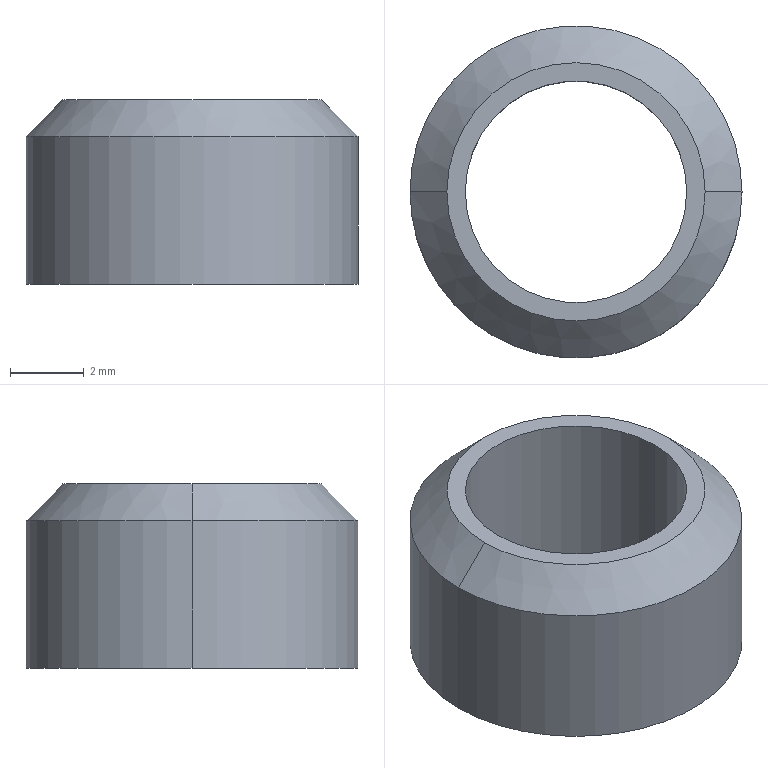Component | SolidWorks | Adjuster-1 | 1 solid | 8 faces | box 9 x 9 x 5 mm | volume 164 mm3 | cylinder 4 | cone 2 | plane 2 | commonest cylinder face diameters 6 x2 9 x2
build123d program:
from build123d import *

# Parameters (mm, degrees)
SKETCH1_R           = 4.5
SKETCH1_R_2         = 3
BOSS_EXTRUDE1_DEPTH = 5
CHAMFER1_SIZE       = 1


with BuildPart() as part:
    # Sketch1 → Boss-Extrude1 (new body)
    with BuildSketch(Plane.XY):
        Circle(SKETCH1_R)
        Circle(SKETCH1_R_2, mode=Mode.SUBTRACT)
    extrude(amount=BOSS_EXTRUDE1_DEPTH)

    # Chamfer1
    chamfer1_edges = [part.edges().sort_by_distance(p)[0] for p in [
        (-4.5, 0, 5),
    ]]
    chamfer(chamfer1_edges, length=CHAMFER1_SIZE)


solid = part.part

# Placed as in the assembly
solid = solid.moved(Location((-218.606, 95.367, 1090.85), (0, 0, 0)))
STEP:
#1=COLOUR_RGB('',0.7922,0.8196,0.9333);
#2=FILL_AREA_STYLE_COLOUR('',#1);
#3=FILL_AREA_STYLE('',(#2));
#4=SURFACE_STYLE_FILL_AREA(#3);
#5=SURFACE_SIDE_STYLE('',(#4));
#6=SURFACE_STYLE_USAGE(.BOTH.,#5);
#7=PRESENTATION_STYLE_ASSIGNMENT((#6));
#8=CARTESIAN_POINT('',(-8.469,3.755,43.144));
#9=VERTEX_POINT('',#8);
#10=CARTESIAN_POINT('',(-8.744,3.755,43.144));
#11=VERTEX_POINT('',#10);
#12=CARTESIAN_POINT('',(-8.607,3.755,43.144));
#13=DIRECTION('',(0.,0.,1.));
#14=DIRECTION('',(1.,0.,0.));
#15=AXIS2_PLACEMENT_3D('',#12,#13,#14);
#16=CIRCLE('',#15,0.1378);
#17=EDGE_CURVE('',#9,#11,#16,.T.);
#18=ORIENTED_EDGE('',*,*,#17,.F.);
#19=CARTESIAN_POINT('',(-8.429,3.755,43.104));
#20=VERTEX_POINT('',#19);
#21=CARTESIAN_POINT('',(-8.469,3.755,43.144));
#22=DIRECTION('',(0.7071,0.,-0.7071));
#23=VECTOR('',#22,39.37);
#24=LINE('',#21,#23);
#25=EDGE_CURVE('',#9,#20,#24,.T.);
#26=ORIENTED_EDGE('',*,*,#25,.T.);
#27=CARTESIAN_POINT('',(-8.784,3.755,43.104));
#28=VERTEX_POINT('',#27);
#29=CARTESIAN_POINT('',(-8.607,3.755,43.104));
#30=DIRECTION('',(0.,0.,-1.));
#31=DIRECTION('',(1.,0.,0.));
#32=AXIS2_PLACEMENT_3D('',#29,#30,#31);
#33=CIRCLE('',#32,0.1772);
#34=EDGE_CURVE('',#28,#20,#33,.T.);
#35=ORIENTED_EDGE('',*,*,#34,.F.);
#36=CARTESIAN_POINT('',(-8.744,3.755,43.144));
#37=DIRECTION('',(-0.7071,0.,-0.7071));
#38=VECTOR('',#37,39.37);
#39=LINE('',#36,#38);
#40=EDGE_CURVE('',#11,#28,#39,.T.);
#41=ORIENTED_EDGE('',*,*,#40,.F.);
#42=EDGE_LOOP('',(#18,#26,#35,#41));
#43=FACE_OUTER_BOUND('',#42,.T.);
#44=CARTESIAN_POINT('',(-8.607,3.755,43.144));
#45=DIRECTION('',(0.,0.,-1.));
#46=DIRECTION('',(-1.,0.,0.));
#47=AXIS2_PLACEMENT_3D('',#44,#45,#46);
#48=CONICAL_SURFACE('',#47,0.1378,0.7854);
#49=ADVANCED_FACE('',(#43),#48,.T.);
#50=CARTESIAN_POINT('',(-8.725,3.755,43.144));
#51=VERTEX_POINT('',#50);
#52=CARTESIAN_POINT('',(-8.488,3.755,43.144));
#53=VERTEX_POINT('',#52);
#54=CARTESIAN_POINT('',(-8.607,3.755,43.144));
#55=DIRECTION('',(0.,0.,1.));
#56=DIRECTION('',(1.,0.,0.));
#57=AXIS2_PLACEMENT_3D('',#54,#55,#56);
#58=CIRCLE('',#57,0.1181);
#59=EDGE_CURVE('',#51,#53,#58,.T.);
#60=ORIENTED_EDGE('',*,*,#59,.T.);
#61=CARTESIAN_POINT('',(-8.488,3.755,42.947));
#62=VERTEX_POINT('',#61);
#63=CARTESIAN_POINT('',(-8.488,3.755,43.144));
#64=DIRECTION('',(0.,0.,-1.));
#65=VECTOR('',#64,39.37);
#66=LINE('',#63,#65);
#67=EDGE_CURVE('',#53,#62,#66,.T.);
#68=ORIENTED_EDGE('',*,*,#67,.T.);
#69=CARTESIAN_POINT('',(-8.725,3.755,42.947));
#70=VERTEX_POINT('',#69);
#71=CARTESIAN_POINT('',(-8.607,3.755,42.947));
#72=DIRECTION('',(0.,0.,1.));
#73=DIRECTION('',(1.,0.,0.));
#74=AXIS2_PLACEMENT_3D('',#71,#72,#73);
#75=CIRCLE('',#74,0.1181);
#76=EDGE_CURVE('',#70,#62,#75,.T.);
#77=ORIENTED_EDGE('',*,*,#76,.F.);
#78=CARTESIAN_POINT('',(-8.725,3.755,43.144));
#79=DIRECTION('',(0.,0.,-1.));
#80=VECTOR('',#79,39.37);
#81=LINE('',#78,#80);
#82=EDGE_CURVE('',#51,#70,#81,.T.);
#83=ORIENTED_EDGE('',*,*,#82,.F.);
#84=EDGE_LOOP('',(#60,#68,#77,#83));
#85=FACE_OUTER_BOUND('',#84,.T.);
#86=CARTESIAN_POINT('',(-8.607,3.755,43.144));
#87=DIRECTION('',(0.,0.,-1.));
#88=DIRECTION('',(-1.,0.,0.));
#89=AXIS2_PLACEMENT_3D('',#86,#87,#88);
#90=CYLINDRICAL_SURFACE('',#89,0.1181);
#91=ADVANCED_FACE('',(#85),#90,.F.);
#92=ORIENTED_EDGE('',*,*,#34,.T.);
#93=CARTESIAN_POINT('',(-8.429,3.755,42.947));
#94=VERTEX_POINT('',#93);
#95=CARTESIAN_POINT('',(-8.429,3.755,43.144));
#96=DIRECTION('',(0.,0.,-1.));
#97=VECTOR('',#96,39.37);
#98=LINE('',#95,#97);
#99=EDGE_CURVE('',#20,#94,#98,.T.);
#100=ORIENTED_EDGE('',*,*,#99,.T.);
#101=CARTESIAN_POINT('',(-8.784,3.755,42.947));
#102=VERTEX_POINT('',#101);
#103=CARTESIAN_POINT('',(-8.607,3.755,42.947));
#104=DIRECTION('',(0.,0.,1.));
#105=DIRECTION('',(1.,0.,0.));
#106=AXIS2_PLACEMENT_3D('',#103,#104,#105);
#107=CIRCLE('',#106,0.1772);
#108=EDGE_CURVE('',#94,#102,#107,.T.);
#109=ORIENTED_EDGE('',*,*,#108,.T.);
#110=CARTESIAN_POINT('',(-8.784,3.755,43.144));
#111=DIRECTION('',(0.,0.,-1.));
#112=VECTOR('',#111,39.37);
#113=LINE('',#110,#112);
#114=EDGE_CURVE('',#28,#102,#113,.T.);
#115=ORIENTED_EDGE('',*,*,#114,.F.);
#116=EDGE_LOOP('',(#92,#100,#109,#115));
#117=FACE_OUTER_BOUND('',#116,.T.);
#118=CARTESIAN_POINT('',(-8.607,3.755,43.144));
#119=DIRECTION('',(0.,0.,-1.));
#120=DIRECTION('',(-1.,0.,0.));
#121=AXIS2_PLACEMENT_3D('',#118,#119,#120);
#122=CYLINDRICAL_SURFACE('',#121,0.1772);
#123=ADVANCED_FACE('',(#117),#122,.T.);
#124=CARTESIAN_POINT('',(-8.607,3.755,43.144));
#125=DIRECTION('',(0.,0.,1.));
#126=DIRECTION('',(1.,0.,0.));
#127=AXIS2_PLACEMENT_3D('',#124,#125,#126);
#128=CIRCLE('',#127,0.1378);
#129=EDGE_CURVE('',#11,#9,#128,.T.);
#130=ORIENTED_EDGE('',*,*,#129,.T.);
#131=ORIENTED_EDGE('',*,*,#17,.T.);
#132=EDGE_LOOP('',(#130,#131));
#133=FACE_OUTER_BOUND('',#132,.T.);
#134=ORIENTED_EDGE('',*,*,#59,.F.);
#135=CARTESIAN_POINT('',(-8.607,3.755,43.144));
#136=DIRECTION('',(0.,0.,1.));
#137=DIRECTION('',(1.,0.,0.));
#138=AXIS2_PLACEMENT_3D('',#135,#136,#137);
#139=CIRCLE('',#138,0.1181);
#140=EDGE_CURVE('',#53,#51,#139,.T.);
#141=ORIENTED_EDGE('',*,*,#140,.F.);
#142=EDGE_LOOP('',(#134,#141));
#143=FACE_BOUND('',#142,.T.);
#144=CARTESIAN_POINT('',(-8.607,3.755,43.144));
#145=DIRECTION('',(0.,0.,1.));
#146=DIRECTION('',(1.,0.,0.));
#147=AXIS2_PLACEMENT_3D('',#144,#145,#146);
#148=PLANE('',#147);
#149=ADVANCED_FACE('',(#133,#143),#148,.T.);
#150=CARTESIAN_POINT('',(-8.607,3.755,42.947));
#151=DIRECTION('',(0.,0.,1.));
#152=DIRECTION('',(1.,0.,0.));
#153=AXIS2_PLACEMENT_3D('',#150,#151,#152);
#154=CIRCLE('',#153,0.1772);
#155=EDGE_CURVE('',#102,#94,#154,.T.);
#156=ORIENTED_EDGE('',*,*,#155,.F.);
#157=ORIENTED_EDGE('',*,*,#108,.F.);
#158=EDGE_LOOP('',(#156,#157));
#159=FACE_OUTER_BOUND('',#158,.T.);
#160=ORIENTED_EDGE('',*,*,#76,.T.);
#161=CARTESIAN_POINT('',(-8.607,3.755,42.947));
#162=DIRECTION('',(0.,0.,1.));
#163=DIRECTION('',(1.,0.,0.));
#164=AXIS2_PLACEMENT_3D('',#161,#162,#163);
#165=CIRCLE('',#164,0.1181);
#166=EDGE_CURVE('',#62,#70,#165,.T.);
#167=ORIENTED_EDGE('',*,*,#166,.T.);
#168=EDGE_LOOP('',(#160,#167));
#169=FACE_BOUND('',#168,.T.);
#170=CARTESIAN_POINT('',(-8.607,3.755,42.947));
#171=DIRECTION('',(0.,0.,1.));
#172=DIRECTION('',(1.,0.,0.));
#173=AXIS2_PLACEMENT_3D('',#170,#171,#172);
#174=PLANE('',#173);
#175=ADVANCED_FACE('',(#159,#169),#174,.F.);
#176=ORIENTED_EDGE('',*,*,#99,.F.);
#177=CARTESIAN_POINT('',(-8.607,3.755,43.104));
#178=DIRECTION('',(0.,0.,-1.));
#179=DIRECTION('',(1.,0.,0.));
#180=AXIS2_PLACEMENT_3D('',#177,#178,#179);
#181=CIRCLE('',#180,0.1772);
#182=EDGE_CURVE('',#20,#28,#181,.T.);
#183=ORIENTED_EDGE('',*,*,#182,.T.);
#184=ORIENTED_EDGE('',*,*,#114,.T.);
#185=ORIENTED_EDGE('',*,*,#155,.T.);
#186=EDGE_LOOP('',(#176,#183,#184,#185));
#187=FACE_OUTER_BOUND('',#186,.T.);
#188=CARTESIAN_POINT('',(-8.607,3.755,43.144));
#189=DIRECTION('',(0.,0.,-1.));
#190=DIRECTION('',(-1.,0.,0.));
#191=AXIS2_PLACEMENT_3D('',#188,#189,#190);
#192=CYLINDRICAL_SURFACE('',#191,0.1772);
#193=ADVANCED_FACE('',(#187),#192,.T.);
#194=ORIENTED_EDGE('',*,*,#67,.F.);
#195=ORIENTED_EDGE('',*,*,#140,.T.);
#196=ORIENTED_EDGE('',*,*,#82,.T.);
#197=ORIENTED_EDGE('',*,*,#166,.F.);
#198=EDGE_LOOP('',(#194,#195,#196,#197));
#199=FACE_OUTER_BOUND('',#198,.T.);
#200=CARTESIAN_POINT('',(-8.607,3.755,43.144));
#201=DIRECTION('',(0.,0.,-1.));
#202=DIRECTION('',(-1.,0.,0.));
#203=AXIS2_PLACEMENT_3D('',#200,#201,#202);
#204=CYLINDRICAL_SURFACE('',#203,0.1181);
#205=ADVANCED_FACE('',(#199),#204,.F.);
#206=ORIENTED_EDGE('',*,*,#25,.F.);
#207=ORIENTED_EDGE('',*,*,#129,.F.);
#208=ORIENTED_EDGE('',*,*,#40,.T.);
#209=ORIENTED_EDGE('',*,*,#182,.F.);
#210=EDGE_LOOP('',(#206,#207,#208,#209));
#211=FACE_OUTER_BOUND('',#210,.T.);
#212=CARTESIAN_POINT('',(-8.607,3.755,43.144));
#213=DIRECTION('',(0.,0.,-1.));
#214=DIRECTION('',(-1.,0.,0.));
#215=AXIS2_PLACEMENT_3D('',#212,#213,#214);
#216=CONICAL_SURFACE('',#215,0.1378,0.7854);
#217=ADVANCED_FACE('',(#211),#216,.T.);
#218=CLOSED_SHELL('',(#49,#91,#123,#149,#175,#193,#205,#217));
#219=MANIFOLD_SOLID_BREP('',#218);
#220=STYLED_ITEM('',(#7),#219);
#221=(LENGTH_UNIT()NAMED_UNIT(*)SI_UNIT($,.METRE.));
#222=LENGTH_MEASURE_WITH_UNIT(LENGTH_MEASURE(0.0254),#221);
#223=DIMENSIONAL_EXPONENTS(1.,0.,0.,0.,0.,0.,0.);
#224=(CONVERSION_BASED_UNIT('',#222)LENGTH_UNIT()NAMED_UNIT(#223));
#225=UNCERTAINTY_MEASURE_WITH_UNIT(LENGTH_MEASURE(0.00001),#224,'','');
#226=(NAMED_UNIT(*)PLANE_ANGLE_UNIT()SI_UNIT($,.RADIAN.));
#227=(NAMED_UNIT(*)SI_UNIT($,.STERADIAN.)SOLID_ANGLE_UNIT());
#228=(GEOMETRIC_REPRESENTATION_CONTEXT(3)GLOBAL_UNCERTAINTY_ASSIGNED_CONTEXT((#225))GLOBAL_UNIT_ASSIGNED_CONTEXT((#224,#226,#227))REPRESENTATION_CONTEXT('',''));
#229=MECHANICAL_DESIGN_GEOMETRIC_PRESENTATION_REPRESENTATION('',(#220),#228);
#230=CARTESIAN_POINT('',(0.,0.,0.));
#231=DIRECTION('',(0.,0.,1.));
#232=DIRECTION('',(1.,0.,0.));
#233=AXIS2_PLACEMENT_3D('',#230,#231,#232);
#234=(LENGTH_UNIT()NAMED_UNIT(*)SI_UNIT($,.METRE.));
#235=LENGTH_MEASURE_WITH_UNIT(LENGTH_MEASURE(0.0254),#234);
#236=DIMENSIONAL_EXPONENTS(1.,0.,0.,0.,0.,0.,0.);
#237=(CONVERSION_BASED_UNIT('',#235)LENGTH_UNIT()NAMED_UNIT(#236));
#238=UNCERTAINTY_MEASURE_WITH_UNIT(LENGTH_MEASURE(0.00001),#237,'','');
#239=(NAMED_UNIT(*)PLANE_ANGLE_UNIT()SI_UNIT($,.RADIAN.));
#240=(NAMED_UNIT(*)SI_UNIT($,.STERADIAN.)SOLID_ANGLE_UNIT());
#241=(GEOMETRIC_REPRESENTATION_CONTEXT(3)GLOBAL_UNCERTAINTY_ASSIGNED_CONTEXT((#238))GLOBAL_UNIT_ASSIGNED_CONTEXT((#237,#239,#240))REPRESENTATION_CONTEXT('',''));
#242=ADVANCED_BREP_SHAPE_REPRESENTATION('',(#219,#233),#241);
#243=PRESENTATION_LAYER_ASSIGNMENT('','',(#220));